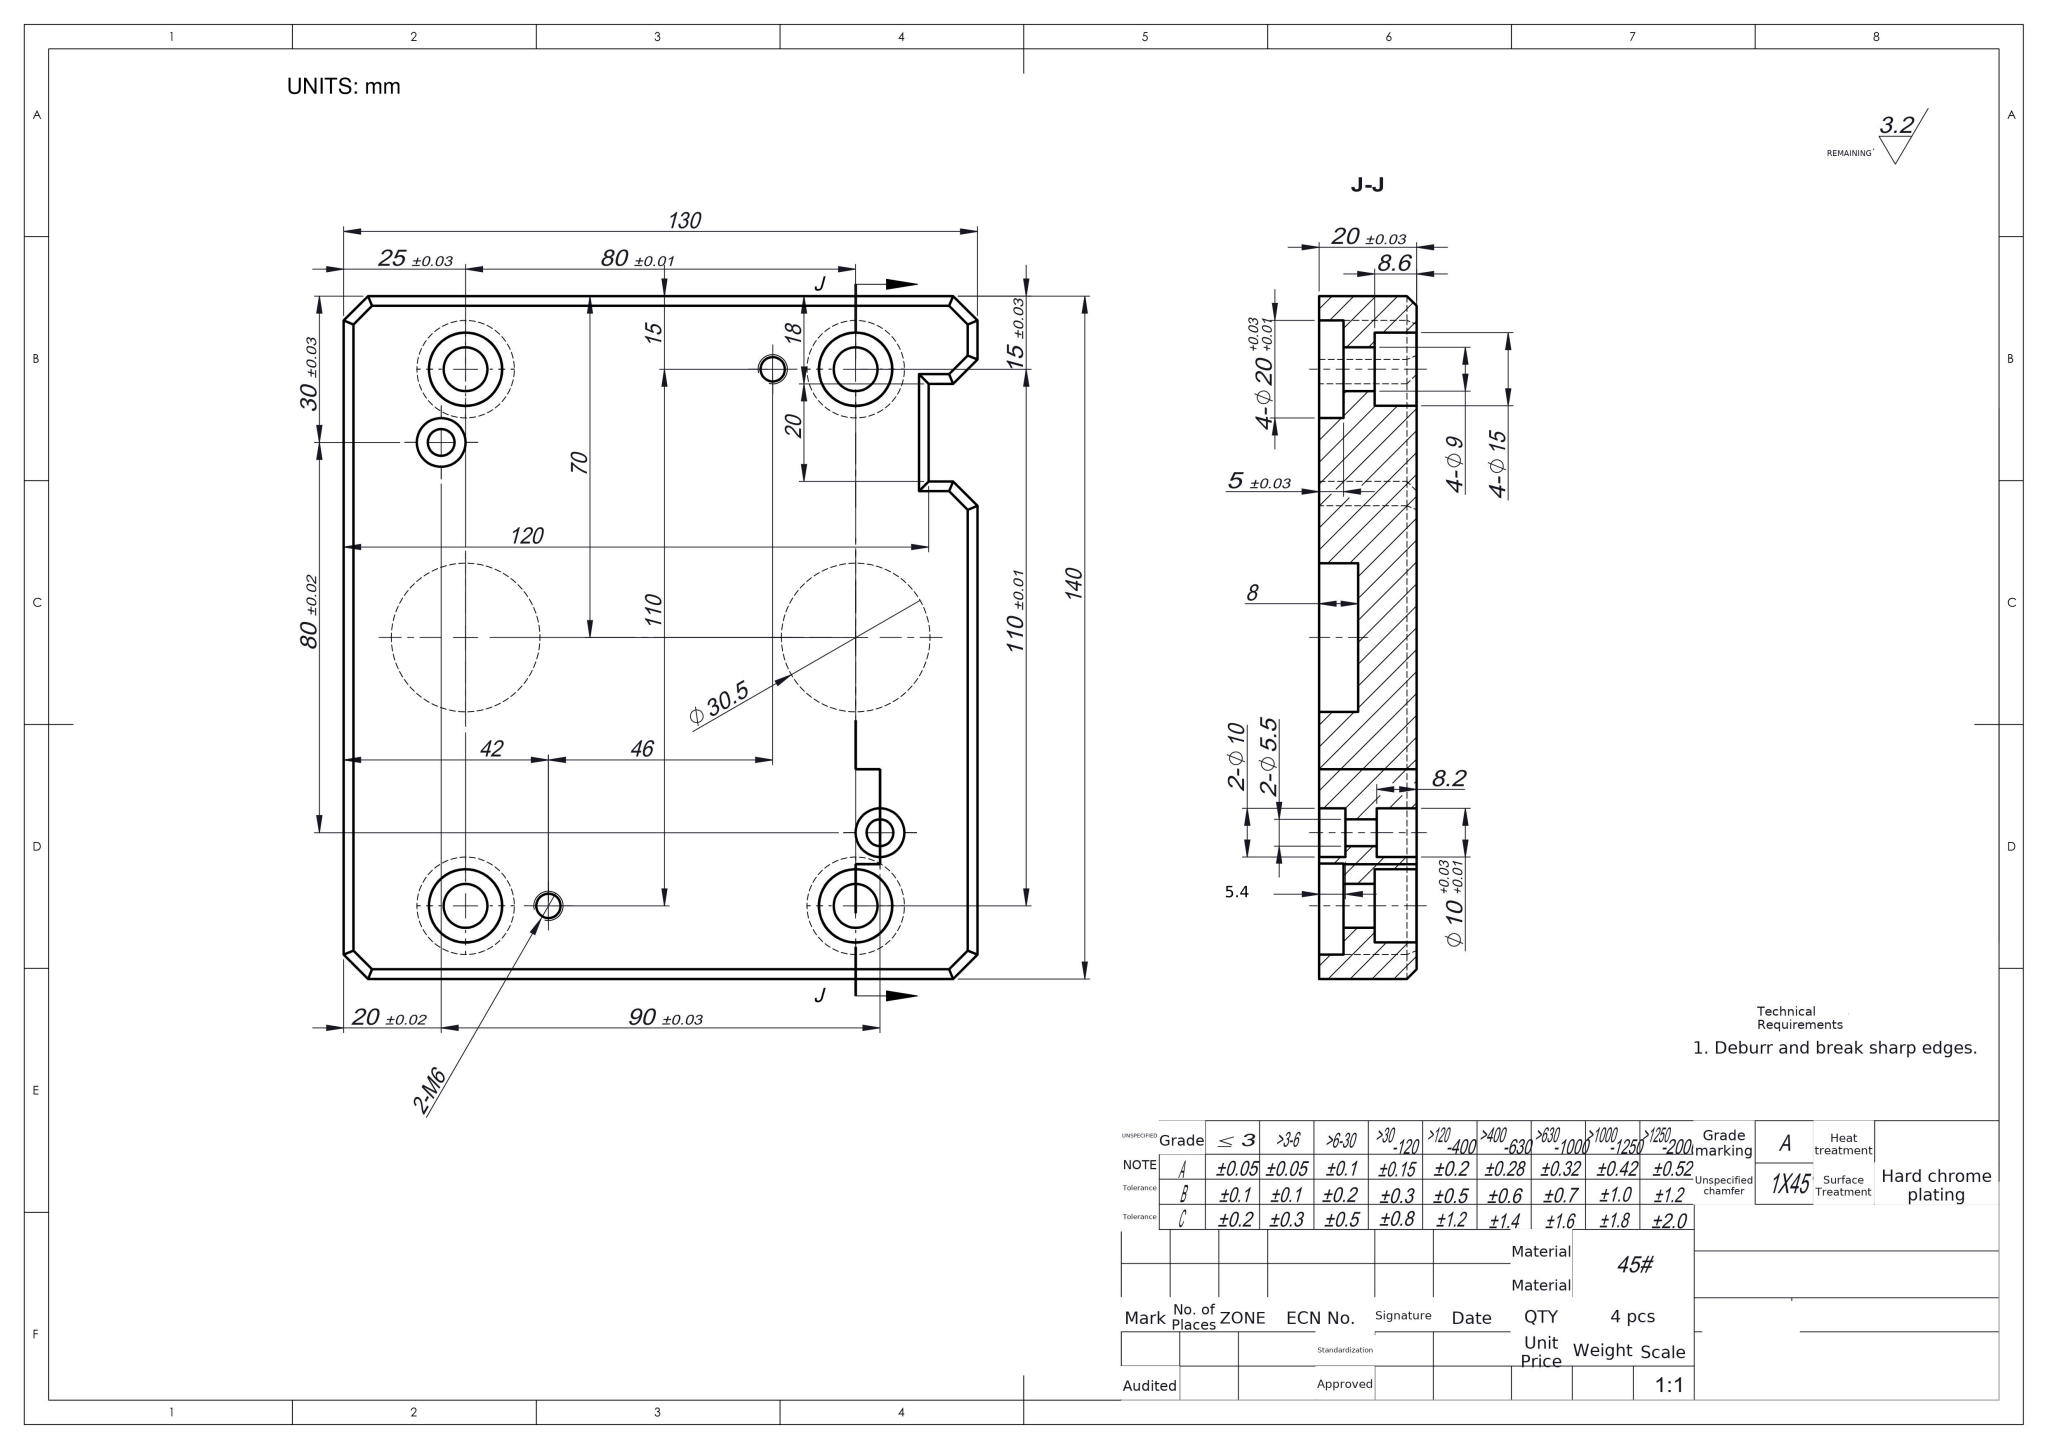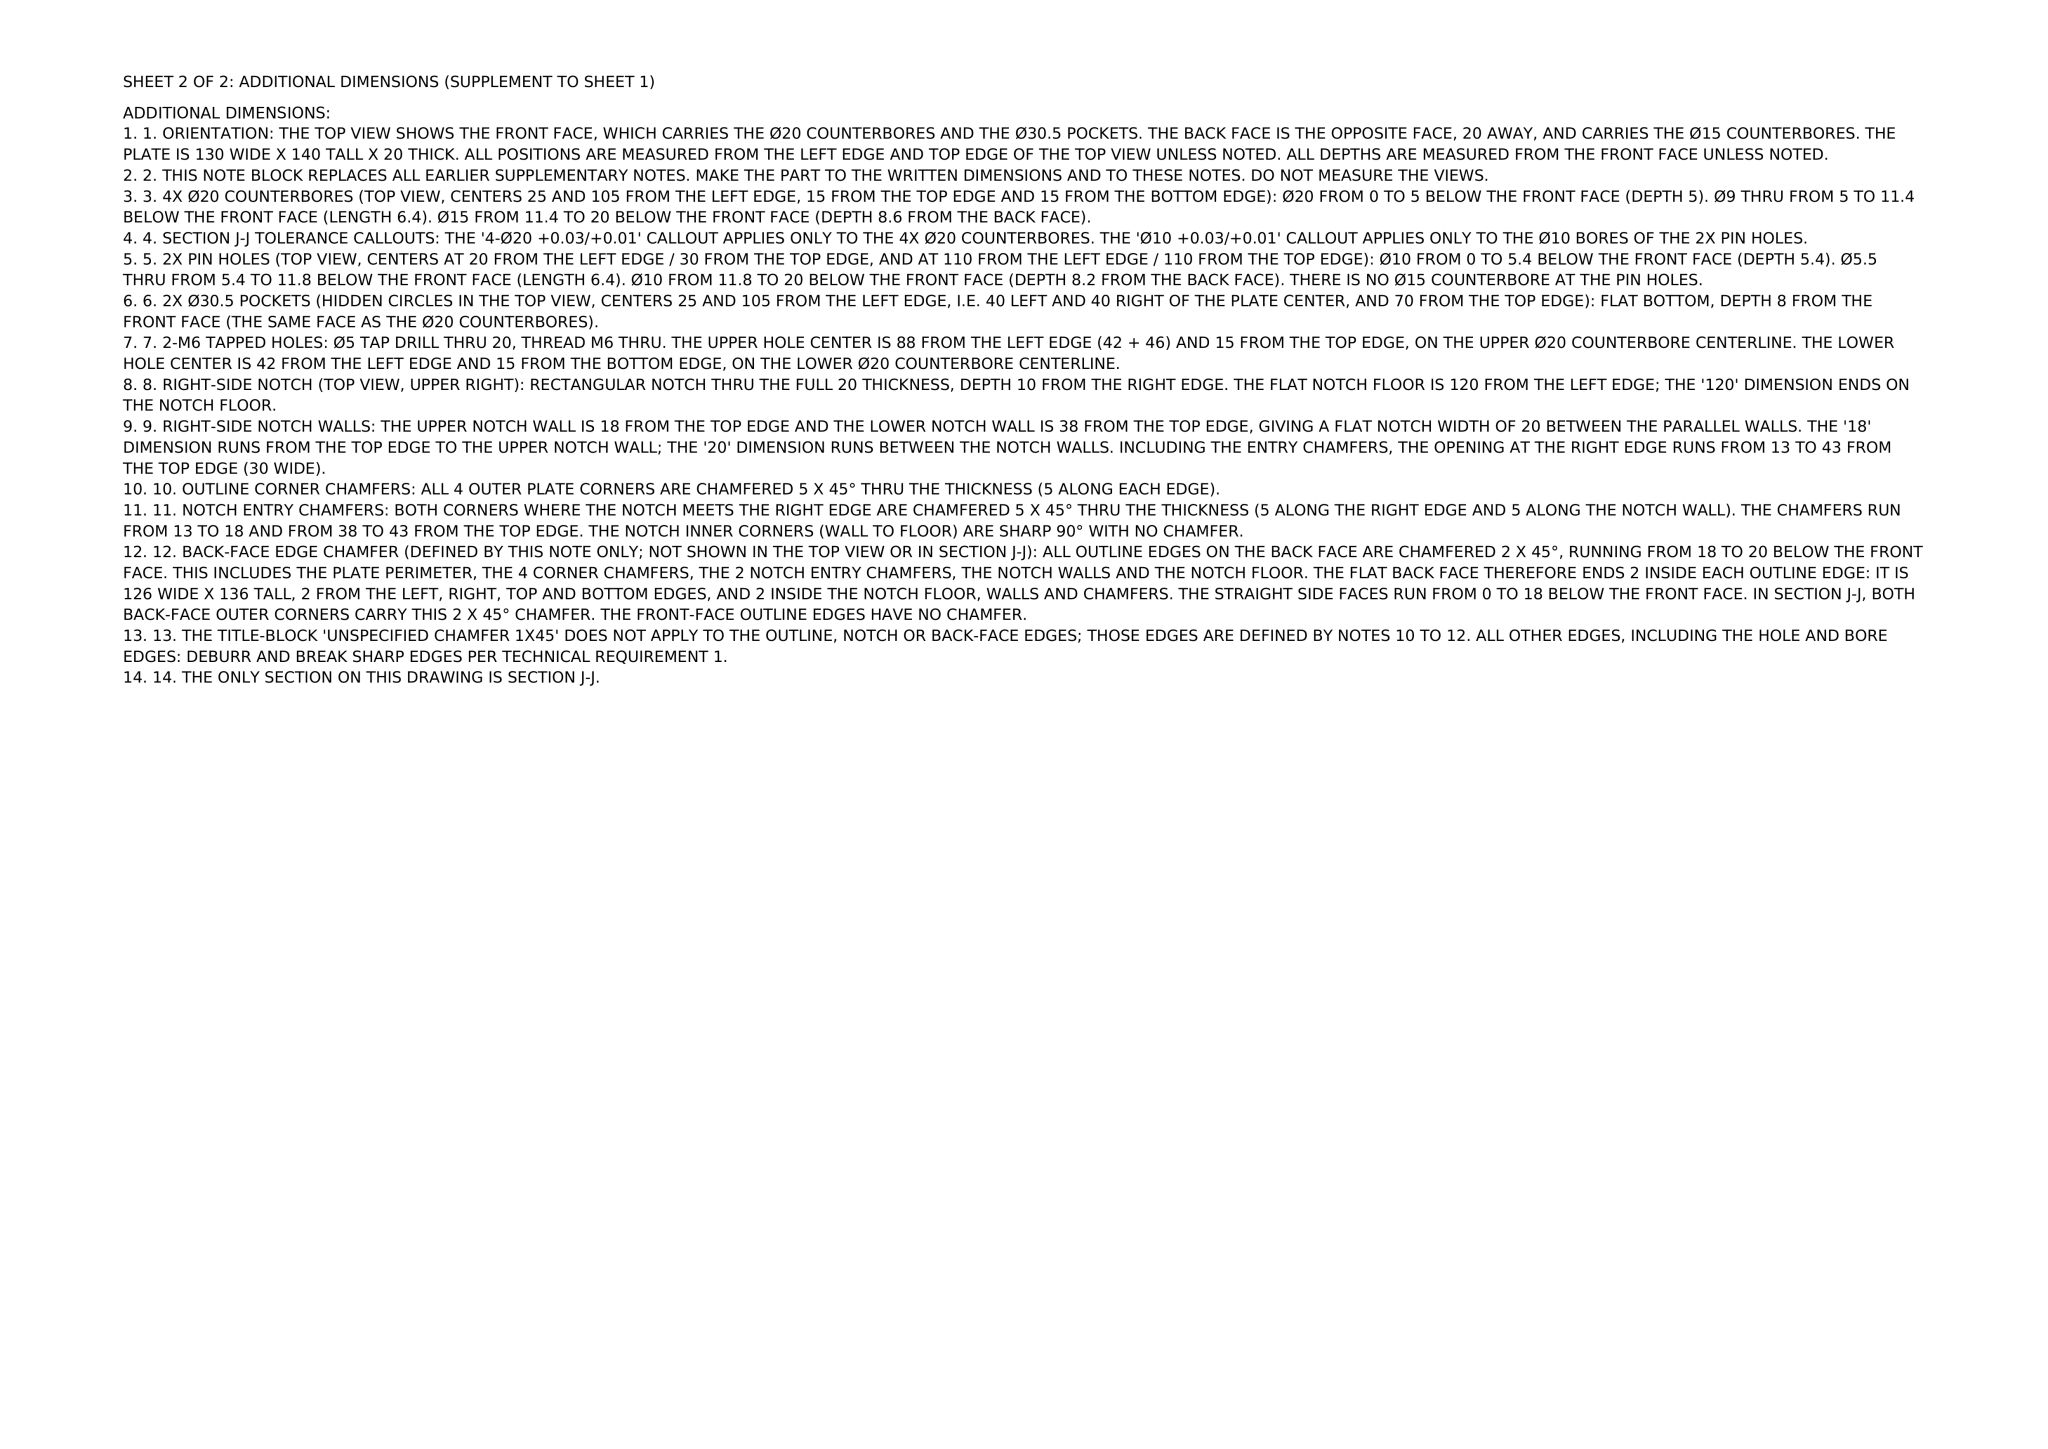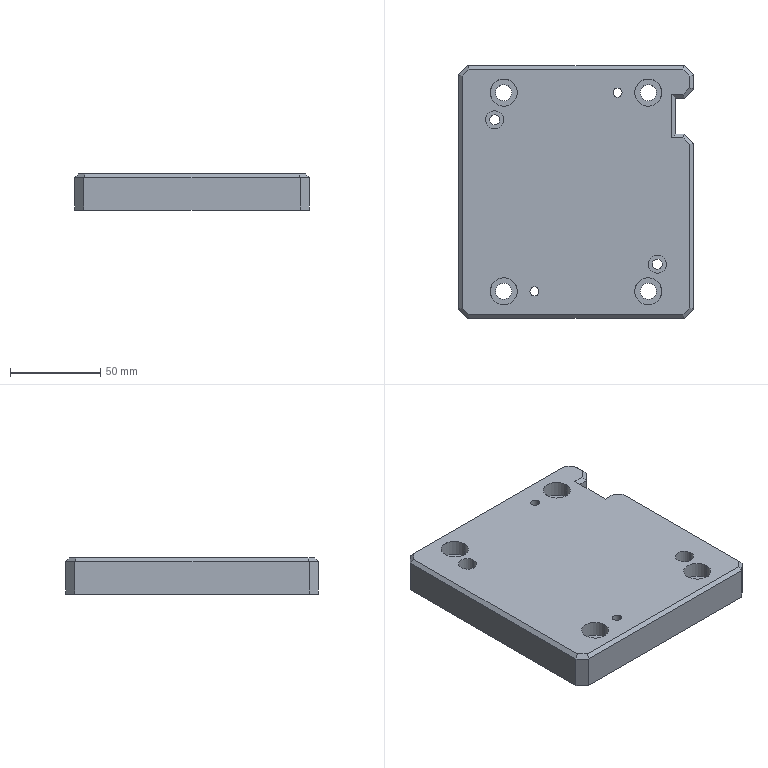Part | NX | mm | 1 solid | 100 faces | box 130 x 140 x 20 mm | volume 328517 mm3 | cylinder 44 | plane 44 | cone 12 | commonest cylinder face diameters 10 x8 20 x8 15 x8 9 x8 5 x4 5.5 x4 30.5 x4